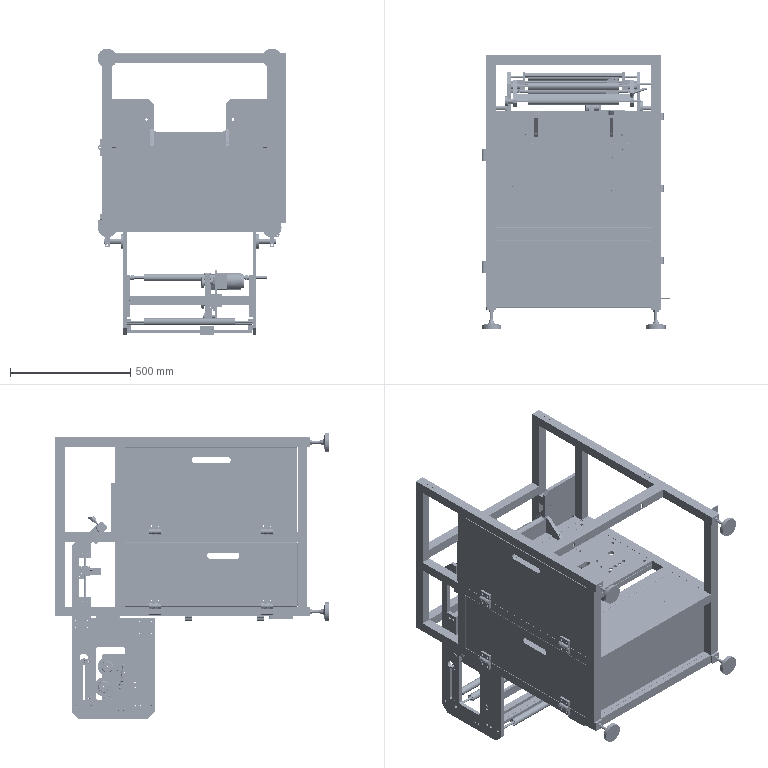Assembly | SolidWorks | mm | 101 component files | 142 solids | 7091 faces | box 785 x 1140 x 1193 mm | volume 25099251 mm3 | plane 4410 | cylinder 1840 | cone 476 | torus 269 | sphere 56 | spline 40 | commonest cylinder face diameters 6 x219 0.4 x172 2 x152 5 x146 10 x115 9 x84 20 x78 7 x78
Bill of materials:
AdjustingScrew | 1 |  | Flanged hollow cylindrical bushing/spacer: a wide, short disc head with a longer, smaller-diameter tubular shank that is coaxial with it. A through bore runs along the axis.
CodingMachine | 1 |  | Multi-body assembly-like geometry: a cylindrical housing with a domed end, mounted on a rectangular block attached to stacked plates. The plates are joined by small rods/standoffs, and several cylindrical bodies (drums/pulleys) sit between and beside the plates. A rectangular box with a window-like cutout projects from one side.
CodingMachineSupport | 1 |  | Long, straight rectangular bar with one small slotted or oblong hole near each end, passing through the bar's wide side.
ConnectingBase | 2 |  | Solid cylindrical shaft with a coaxial circular flange at one end. The flange has four through holes evenly spaced on a bolt circle.
ConnectingPlate | 1 |  | Long, thin rectangular strip/bar with two small holes near each end (four holes in total) on one face.
Cover | 1 |  | Flat rectangular (near-square) plate with four corner through holes and one larger central through hole.
FilmConnectionPlate | 1 |  | Long U-shaped channel with thin walls: a flat base with two upright side walls and rounded inner/outer bends. There is one small hole near each end of the base and a thin line running along the base.
FilmGuideRodAxis | 1 |  | Long, slender, plain cylindrical rod with flat ends.
FixedSeat | 2 |  | T-shaped block (shaft-support-like): a rectangular top bar with two vertical through holes, and a lower body with a large horizontal bore. A narrow slit runs from the bore to the bottom face, and a cross hole passes through the split portion, consistent with a clamp feature.
Gear | 2 |  | Hollow cylindrical gear/pinion-like part: a smooth cylindrical hub, a short reduced-diameter neck, and a section with straight axial teeth. A through bore runs along the axis, and there is a radial hole in the hub.
HorizontalSidePlate(1) | 1 |  | Flat, elongated plate with a C-shaped profile: a deep rectangular notch along one long edge, a chamfered corner at the top, and a larger hole in the upper section. There are several small holes in the upper and lower sections, and a small step at the lower end.
HorizontalSidePlate(2) | 1 |  | Flat, elongated C-profile plate, nearly identical to unnamed part: a rectangular side notch, a chamfered top corner, a large upper hole, and several small holes. Its lower-end step sits on the opposite side, and the bottom portion looks narrower in the isometric view.
LargeSidePlate(1) | 1 |  | Flat rectangular plate with a large rounded-rectangle through-window, a keyhole-shaped slot (circular hole joined to a long narrow slot), two chamfered bottom corners, many small holes, and shallow stepped recesses along the top edge.
LargeSidePlate(2) | 1 |  | Flat rectangular plate with a large rounded-rectangle through-window, a keyhole-shaped slot, two chamfered bottom corners, many small holes, and small notches/steps at the top edge and upper left edge.
LeftSupportBlock | 1 |  | Elongated flat link-like bar with chamfered (clipped) corners, a smaller through-hole near one end and a larger through-hole near the other, plus small cross holes through the side edge.
LongGearAxis | 1 |  | Long slender solid cylindrical rod with plain ends; the end view shows a faceted circular profile with a small edge chamfer or bevel.
M5AdjustableHandle | 1 |  | Clamping-lever-style component: a cylindrical hub with a tapered lever arm, a hexagonal section below the hub, and a smaller cylindrical stud/pin coming out of the bottom. The top of the hub has a shallow recess with a cross-shaped mark.
NameDuplicate-1Crossbar | 1 |  | Long rectangular flat bar with one small oblong hole or slot near each end.
NameDuplicate-1SupportBlock | 6 |  | Rectangular block with one through-hole in one face direction and two parallel through-holes in a perpendicular direction.
PhotoelectricBracket | 1 |  | Bracket made of a flat plate with a long slot and two round holes, joined at one end to a thicker block that has a transverse bore and a split slit through the bore (split-clamp-style geometry).
PhotoelectricSensor | 1 |  | Rectangular housing-like block with stepped and angled outer profile, a knurled cylindrical knob at one end, two holes on the top face, and two small cylindrical protrusions on one side face.
PhotoelectricSlideRod | 2 |  | Slender solid cylindrical rod or pin with plain ends; the end view shows a circular profile with a faceted outer chamfer band.
Rack | 2 |  | Long rectangular bar with a row of small sawtooth/serrated teeth along one narrow edge and an oblong slot near each end.
RightSupportBlock | 1 |  | Elongated flat link-like bar with chamfered corners, a small through-hole near one end and a large through-hole near the other, plus three small holes on the narrow edge and one hole on another edge face.
Roller1-1 | 1 |  | Long straight round tube with a uniform annular cross-section and plain square-cut ends.
Roller1 | 5 |  | Long straight round tube with a uniform annular cross-section and plain ends. Very similar to unnamed part.
RollerAxis1 | 3 |  | Very slender round rod or tube with an axial bore at the end. Faint lines near each end may mark short end features.
RollerAxis3 | 1 |  | Long, slender, solid cylindrical rod with flat ends.
RubberFrame | 1 |  | Rectangular block with a wide rectangular U-shaped channel cut through its underside along one axis, forming an inverted-U profile. One long side face has two small holes.
RubberPlate | 1 |  | Flat, thin rectangular plate with no visible holes or features.
RubberPlateBaffle | 2 |  | Long L-shaped angle with unequal legs. The wider leg has two round through holes near its ends.
SCLinearBearing | 2 |  | Rectangular block with a large round bore through its top face, four small through holes in a rectangular pattern on one side face, and one cross hole on an adjacent face.
SmallHandwheel | 2 |  | Headed cylindrical pin: a short, larger-diameter disc head on a smaller, longer cylindrical shank. The head's outer face is slightly domed.
SmoothRod | 4 |  | Very slender straight round tube or rod with a small axial bore at the end.
SupportAxis | 2 |  | Cylindrical sleeve or bushing with a central axial bore and one narrow, shallow circumferential groove near mid-length on the outside diameter.
SupportBase | 4 |  | Rectangular block with two chamfered corners at one end, a large through hole near that end, and two small holes in one narrow side face.
SupportPlate_2 | 2 |  | Thick rectangular plate with a smaller rectangular tab sticking out from the middle of one long edge, pierced by eight round through-holes.
FootCup | 4 |  | Round disc base with a chamfered upper edge. A flared, filleted neck rises from it into a slender cylindrical shaft with a hex nut partway along and a chamfered free end.
FormerSupportPlate | 1 |  | Thin flat plate with a wide, deep rectangular U-shaped notch cut from the middle of one long edge. The outer corners at the notch are chamfered, the inner notch corners are filleted, and there are twelve small round holes.
AnchorThreadPlate | 4 |  | Thick square plate with rounded corners and a single central round through-hole. The hole edge is chamfered or rounded.
BottomThinPlate | 1 |  | Plain thin rectangular flat plate or panel with no visible holes or cut-outs.
Frame | 1 |  | Open box-like welded or assembled frame built from square-section tube members. It has a stepped (L-shaped) outline in side view, intermediate horizontal rails and vertical posts, and small cylindrical protrusions along one bottom edge.
FrontBendPlate | 1 |  | Long, thin-walled U-shaped (channel) profile with rounded outer bends and two elongated slots in one side wall.
FrontLowerThinPlate | 1 |  | Flat rectangular plate with four small round through-holes in a rectangular pattern.
LowerBendPlate | 1 |  | Long, thin-walled U-shaped channel with rounded outer bends and no visible holes or slots.
MiddleBendPlate | 1 |  | Long, shallow U-shaped channel with rounded outer bends and three small round holes spaced along the centreline of the web.
MiddleThinPlate | 1 |  | Plain thin rectangular flat plate or panel with no visible holes or cut-outs.
MountingPlate | 4 |  | Rectangular plate with rounded corners, two round holes near the ends with chamfered edges, and a shallow rectangular step pocket cut into one long edge.
RearThinPlate | 1 |  | Thin flat square plate with two small round through-holes, one near a corner and one inset near the opposite side.
SupportPlate | 2 |  | Long, narrow L-section (angle) strip with a single round hole centred on one leg.
UpperBendPlate | 1 |  | Long L-section (angle) strip with a row of holes along one leg: single holes at each end and the centre, and two pairs of holes placed between them.
Hinge | 8 |  | Block-shaped clevis/knuckle bracket: a rectangular base plate with two mounting holes, and two spaced lugs with rounded tops and aligned cross-holes, separated by a slot.
LeftGlassDoor | 1 |  | Thin flat rectangular panel with one elongated slot (rounded ends) near the top centre and two pairs of small holes near the bottom corners.
LongitudinalSealPanel | 1 |  | Thick flat rectangular mounting plate with a dense, roughly mirror-symmetric hole pattern: two central obround slots, two circular bolt-circle-like hole groups, rows of larger holes, perimeter holes, and one larger isolated hole.
SideDoor | 1 |  | Rectangular panel with short perimeter flanges or bevelled edges (mitred corners visible), one obround slot near the top centre, and two pairs of small holes near the bottom corners.
SupportBlock | 2 |  | Prismatic wedge or gusset block: a roughly right-triangular/trapezoidal profile with an inclined face, a small rectangular step notch at the bottom, and one round hole.
Mates:
1. coincident | PhotoelectricBracket-1 face at (185.293, 491.5, -185.544) dir (0, -1, 0) | PhotoelectricSensor-1 face at (207.293, 491.5, -181.003) dir (0, -1, 0)
2. coincident | PhotoelectricBracket-1 face at (185.293, 586.5, -185.544) dir (1, 0, 0) | PhotoelectricSensor-1 face at (185.293, 491.5, -181.003) dir (-1, 0, 0)